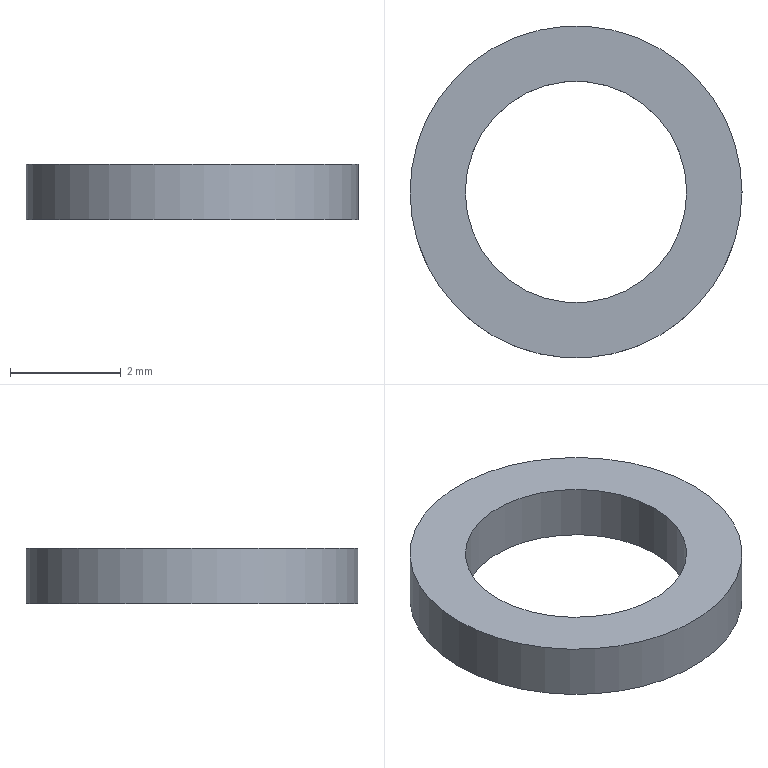Component | NX | SMALL_WASHER | 1 solid | 4 faces | box 6 x 6 x 1 mm | volume 16 mm3 | cylinder 2 | plane 2 | commonest cylinder face diameters 6 x1 4 x1
STEP:
#1=CARTESIAN_POINT('',(0.,0.,0.));
#2=DIRECTION('',(0.,0.,1.));
#3=DIRECTION('',(1.,0.,0.));
#4=AXIS2_PLACEMENT_3D('',#1,#2,#3);
#5=CARTESIAN_POINT('',(16.994,-107.616,12.));
#6=VERTEX_POINT('',#5);
#7=CARTESIAN_POINT('',(13.994,-107.616,12.));
#8=DIRECTION('',(0.,0.,1.));
#9=DIRECTION('',(1.,0.,0.));
#10=AXIS2_PLACEMENT_3D('',#7,#8,#9);
#11=CIRCLE('',#10,3.);
#12=CARTESIAN_POINT('',(13.994,-107.616,12.));
#13=DIRECTION('',(0.,0.,-1.));
#14=DIRECTION('',(0.,1.,0.));
#15=AXIS2_PLACEMENT_3D('',#12,#13,#14);
#16=CYLINDRICAL_SURFACE('',#15,3.);
#17=CARTESIAN_POINT('',(7.854,0.));
#18=DIRECTION('',(-1.,0.));
#19=VECTOR('',#18,1.);
#20=LINE('',#17,#19);
#21=(GEOMETRIC_REPRESENTATION_CONTEXT(2)PARAMETRIC_REPRESENTATION_CONTEXT()REPRESENTATION_CONTEXT('',''));
#22=DEFINITIONAL_REPRESENTATION('',(#20),#21);
#23=PCURVE('',#16,#22);
#24=CARTESIAN_POINT('',(13.994,-107.616,12.));
#25=DIRECTION('',(0.,0.,1.));
#26=DIRECTION('',(0.,-1.,0.));
#27=AXIS2_PLACEMENT_3D('',#24,#25,#26);
#28=PLANE('',#27);
#29=CARTESIAN_POINT('',(0.,0.));
#30=DIRECTION('',(0.,1.));
#31=AXIS2_PLACEMENT_2D('',#29,#30);
#32=CIRCLE('',#31,3.);
#33=(GEOMETRIC_REPRESENTATION_CONTEXT(2)PARAMETRIC_REPRESENTATION_CONTEXT()REPRESENTATION_CONTEXT('',''));
#34=DEFINITIONAL_REPRESENTATION('',(#32),#33);
#35=PCURVE('',#28,#34);
#36=SURFACE_CURVE('',#11,(#23,#35),.PCURVE_S1.);
#37=EDGE_CURVE('',#6,#6,#36,.T.);
#38=ORIENTED_EDGE('',*,*,#37,.F.);
#39=CARTESIAN_POINT('',(16.994,-107.616,11.));
#40=VERTEX_POINT('',#39);
#41=CARTESIAN_POINT('',(16.994,-107.616,12.));
#42=CARTESIAN_POINT('',(16.994,-107.616,11.));
#43=B_SPLINE_CURVE_WITH_KNOTS('',1,(#41,#42),.UNSPECIFIED.,.F.,.F.,(2,2),(0.,1.),.PIECEWISE_BEZIER_KNOTS.);
#44=CARTESIAN_POINT('',(7.854,0.));
#45=DIRECTION('',(0.,1.));
#46=VECTOR('',#45,1.);
#47=LINE('',#44,#46);
#48=(GEOMETRIC_REPRESENTATION_CONTEXT(2)PARAMETRIC_REPRESENTATION_CONTEXT()REPRESENTATION_CONTEXT('',''));
#49=DEFINITIONAL_REPRESENTATION('',(#47),#48);
#50=PCURVE('',#16,#49);
#51=CARTESIAN_POINT('',(1.571,0.));
#52=DIRECTION('',(0.,1.));
#53=VECTOR('',#52,1.);
#54=LINE('',#51,#53);
#55=(GEOMETRIC_REPRESENTATION_CONTEXT(2)PARAMETRIC_REPRESENTATION_CONTEXT()REPRESENTATION_CONTEXT('',''));
#56=DEFINITIONAL_REPRESENTATION('',(#54),#55);
#57=PCURVE('',#16,#56);
#58=SEAM_CURVE('',#43,(#50,#57),.PCURVE_S1.);
#59=EDGE_CURVE('',#6,#40,#58,.T.);
#60=ORIENTED_EDGE('',*,*,#59,.T.);
#61=CARTESIAN_POINT('',(13.994,-107.616,11.));
#62=DIRECTION('',(0.,0.,1.));
#63=DIRECTION('',(1.,0.,0.));
#64=AXIS2_PLACEMENT_3D('',#61,#62,#63);
#65=CIRCLE('',#64,3.);
#66=CARTESIAN_POINT('',(7.854,1.));
#67=DIRECTION('',(-1.,0.));
#68=VECTOR('',#67,1.);
#69=LINE('',#66,#68);
#70=(GEOMETRIC_REPRESENTATION_CONTEXT(2)PARAMETRIC_REPRESENTATION_CONTEXT()REPRESENTATION_CONTEXT('',''));
#71=DEFINITIONAL_REPRESENTATION('',(#69),#70);
#72=PCURVE('',#16,#71);
#73=CARTESIAN_POINT('',(13.994,-107.616,11.));
#74=DIRECTION('',(0.,0.,1.));
#75=DIRECTION('',(0.,-1.,0.));
#76=AXIS2_PLACEMENT_3D('',#73,#74,#75);
#77=PLANE('',#76);
#78=CARTESIAN_POINT('',(0.,0.));
#79=DIRECTION('',(0.,1.));
#80=AXIS2_PLACEMENT_2D('',#78,#79);
#81=CIRCLE('',#80,3.);
#82=(GEOMETRIC_REPRESENTATION_CONTEXT(2)PARAMETRIC_REPRESENTATION_CONTEXT()REPRESENTATION_CONTEXT('',''));
#83=DEFINITIONAL_REPRESENTATION('',(#81),#82);
#84=PCURVE('',#77,#83);
#85=SURFACE_CURVE('',#65,(#72,#84),.PCURVE_S1.);
#86=EDGE_CURVE('',#40,#40,#85,.T.);
#87=ORIENTED_EDGE('',*,*,#86,.T.);
#88=ORIENTED_EDGE('',*,*,#59,.F.);
#89=EDGE_LOOP('',(#38,#60,#87,#88));
#90=FACE_BOUND('',#89,.T.);
#91=ADVANCED_FACE('',(#90),#16,.T.);
#92=CARTESIAN_POINT('',(15.994,-107.616,12.));
#93=VERTEX_POINT('',#92);
#94=CARTESIAN_POINT('',(13.994,-107.616,12.));
#95=DIRECTION('',(0.,0.,1.));
#96=DIRECTION('',(1.,0.,0.));
#97=AXIS2_PLACEMENT_3D('',#94,#95,#96);
#98=CIRCLE('',#97,2.);
#99=CARTESIAN_POINT('',(13.994,-107.616,12.));
#100=DIRECTION('',(0.,0.,-1.));
#101=DIRECTION('',(0.,1.,0.));
#102=AXIS2_PLACEMENT_3D('',#99,#100,#101);
#103=CYLINDRICAL_SURFACE('',#102,2.);
#104=CARTESIAN_POINT('',(7.854,0.));
#105=DIRECTION('',(-1.,0.));
#106=VECTOR('',#105,1.);
#107=LINE('',#104,#106);
#108=(GEOMETRIC_REPRESENTATION_CONTEXT(2)PARAMETRIC_REPRESENTATION_CONTEXT()REPRESENTATION_CONTEXT('',''));
#109=DEFINITIONAL_REPRESENTATION('',(#107),#108);
#110=PCURVE('',#103,#109);
#111=CARTESIAN_POINT('',(0.,0.));
#112=DIRECTION('',(0.,1.));
#113=AXIS2_PLACEMENT_2D('',#111,#112);
#114=CIRCLE('',#113,2.);
#115=(GEOMETRIC_REPRESENTATION_CONTEXT(2)PARAMETRIC_REPRESENTATION_CONTEXT()REPRESENTATION_CONTEXT('',''));
#116=DEFINITIONAL_REPRESENTATION('',(#114),#115);
#117=PCURVE('',#28,#116);
#118=SURFACE_CURVE('',#98,(#110,#117),.PCURVE_S1.);
#119=EDGE_CURVE('',#93,#93,#118,.T.);
#120=ORIENTED_EDGE('',*,*,#119,.F.);
#121=CARTESIAN_POINT('',(15.994,-107.616,11.));
#122=VERTEX_POINT('',#121);
#123=CARTESIAN_POINT('',(15.994,-107.616,12.));
#124=CARTESIAN_POINT('',(15.994,-107.616,11.));
#125=B_SPLINE_CURVE_WITH_KNOTS('',1,(#123,#124),.UNSPECIFIED.,.F.,.F.,(2,2),(0.,1.),.PIECEWISE_BEZIER_KNOTS.);
#126=CARTESIAN_POINT('',(7.854,0.));
#127=DIRECTION('',(0.,1.));
#128=VECTOR('',#127,1.);
#129=LINE('',#126,#128);
#130=(GEOMETRIC_REPRESENTATION_CONTEXT(2)PARAMETRIC_REPRESENTATION_CONTEXT()REPRESENTATION_CONTEXT('',''));
#131=DEFINITIONAL_REPRESENTATION('',(#129),#130);
#132=PCURVE('',#103,#131);
#133=CARTESIAN_POINT('',(1.571,0.));
#134=DIRECTION('',(0.,1.));
#135=VECTOR('',#134,1.);
#136=LINE('',#133,#135);
#137=(GEOMETRIC_REPRESENTATION_CONTEXT(2)PARAMETRIC_REPRESENTATION_CONTEXT()REPRESENTATION_CONTEXT('',''));
#138=DEFINITIONAL_REPRESENTATION('',(#136),#137);
#139=PCURVE('',#103,#138);
#140=SEAM_CURVE('',#125,(#132,#139),.PCURVE_S1.);
#141=EDGE_CURVE('',#93,#122,#140,.T.);
#142=ORIENTED_EDGE('',*,*,#141,.T.);
#143=CARTESIAN_POINT('',(13.994,-107.616,11.));
#144=DIRECTION('',(0.,0.,1.));
#145=DIRECTION('',(1.,0.,0.));
#146=AXIS2_PLACEMENT_3D('',#143,#144,#145);
#147=CIRCLE('',#146,2.);
#148=CARTESIAN_POINT('',(7.854,1.));
#149=DIRECTION('',(-1.,0.));
#150=VECTOR('',#149,1.);
#151=LINE('',#148,#150);
#152=(GEOMETRIC_REPRESENTATION_CONTEXT(2)PARAMETRIC_REPRESENTATION_CONTEXT()REPRESENTATION_CONTEXT('',''));
#153=DEFINITIONAL_REPRESENTATION('',(#151),#152);
#154=PCURVE('',#103,#153);
#155=CARTESIAN_POINT('',(0.,0.));
#156=DIRECTION('',(0.,1.));
#157=AXIS2_PLACEMENT_2D('',#155,#156);
#158=CIRCLE('',#157,2.);
#159=(GEOMETRIC_REPRESENTATION_CONTEXT(2)PARAMETRIC_REPRESENTATION_CONTEXT()REPRESENTATION_CONTEXT('',''));
#160=DEFINITIONAL_REPRESENTATION('',(#158),#159);
#161=PCURVE('',#77,#160);
#162=SURFACE_CURVE('',#147,(#154,#161),.PCURVE_S1.);
#163=EDGE_CURVE('',#122,#122,#162,.T.);
#164=ORIENTED_EDGE('',*,*,#163,.T.);
#165=ORIENTED_EDGE('',*,*,#141,.F.);
#166=EDGE_LOOP('',(#120,#142,#164,#165));
#167=FACE_BOUND('',#166,.F.);
#168=ADVANCED_FACE('',(#167),#103,.F.);
#169=ORIENTED_EDGE('',*,*,#37,.T.);
#170=EDGE_LOOP('',(#169));
#171=FACE_BOUND('',#170,.T.);
#172=ORIENTED_EDGE('',*,*,#119,.F.);
#173=EDGE_LOOP('',(#172));
#174=FACE_BOUND('',#173,.T.);
#175=ADVANCED_FACE('',(#171,#174),#28,.T.);
#176=ORIENTED_EDGE('',*,*,#86,.F.);
#177=EDGE_LOOP('',(#176));
#178=FACE_BOUND('',#177,.T.);
#179=ORIENTED_EDGE('',*,*,#163,.T.);
#180=EDGE_LOOP('',(#179));
#181=FACE_BOUND('',#180,.T.);
#182=ADVANCED_FACE('',(#178,#181),#77,.F.);
#183=CLOSED_SHELL('',(#91,#168,#175,#182));
#184=MANIFOLD_SOLID_BREP('',#183);
#185=(LENGTH_UNIT()NAMED_UNIT(*)SI_UNIT(.MILLI.,.METRE.));
#186=UNCERTAINTY_MEASURE_WITH_UNIT(LENGTH_MEASURE(0.00001),#185,'','');
#187=(NAMED_UNIT(*)PLANE_ANGLE_UNIT()SI_UNIT($,.RADIAN.));
#188=(NAMED_UNIT(*)SI_UNIT($,.STERADIAN.)SOLID_ANGLE_UNIT());
#189=(GEOMETRIC_REPRESENTATION_CONTEXT(3)GLOBAL_UNCERTAINTY_ASSIGNED_CONTEXT((#186))GLOBAL_UNIT_ASSIGNED_CONTEXT((#185,#187,#188))REPRESENTATION_CONTEXT('',''));
#190=ADVANCED_BREP_SHAPE_REPRESENTATION('',(#4,#184),#189);